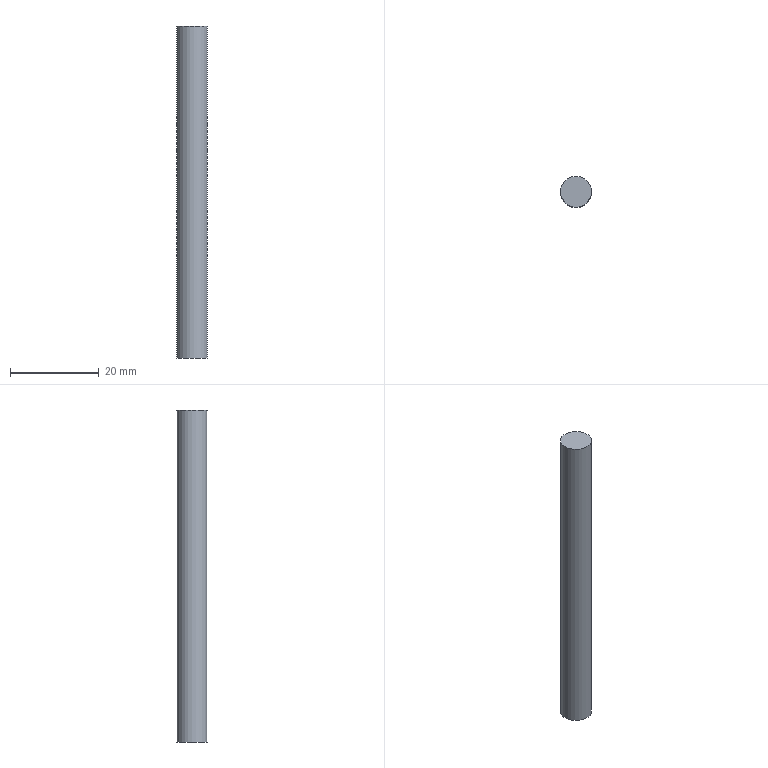Component | NX | SCREW_ROD_2 | 1 solid | 3 faces | box 6.99 x 6.99 x 75 mm | volume 2874 mm3 | plane 2 | cylinder 1 | commonest cylinder face diameters 6.985 x1
STEP:
#1=CARTESIAN_POINT('',(0.,0.,0.));
#2=DIRECTION('',(0.,0.,1.));
#3=DIRECTION('',(1.,0.,0.));
#4=AXIS2_PLACEMENT_3D('',#1,#2,#3);
#5=CARTESIAN_POINT('',(245.993,-0.,-15.));
#6=VERTEX_POINT('',#5);
#7=CARTESIAN_POINT('',(242.5,-0.,-15.));
#8=DIRECTION('',(0.,0.,-1.));
#9=DIRECTION('',(1.,0.,0.));
#10=AXIS2_PLACEMENT_3D('',#7,#8,#9);
#11=CIRCLE('',#10,3.493);
#12=CARTESIAN_POINT('',(242.5,-0.,-15.));
#13=DIRECTION('',(0.,0.,1.));
#14=DIRECTION('',(1.,0.,0.));
#15=AXIS2_PLACEMENT_3D('',#12,#13,#14);
#16=PLANE('',#15);
#17=CARTESIAN_POINT('',(3.493,0.));
#18=CARTESIAN_POINT('',(3.493,-6.049));
#19=CARTESIAN_POINT('',(-1.746,-3.025));
#20=CARTESIAN_POINT('',(-6.985,-0.));
#21=CARTESIAN_POINT('',(-1.746,3.025));
#22=CARTESIAN_POINT('',(3.493,6.049));
#23=CARTESIAN_POINT('',(3.493,0.));
#24=(BOUNDED_CURVE()B_SPLINE_CURVE(2,(#17,#18,#19,#20,#21,#22,#23),.UNSPECIFIED.,.T.,.F.)B_SPLINE_CURVE_WITH_KNOTS((1,2,2,2,2,1),(-2.094,0.,2.094,4.189,6.283,8.378),.UNSPECIFIED.)CURVE()GEOMETRIC_REPRESENTATION_ITEM()RATIONAL_B_SPLINE_CURVE((1.,0.5,1.,0.5,1.,0.5,1.))REPRESENTATION_ITEM(''));
#25=(GEOMETRIC_REPRESENTATION_CONTEXT(2)PARAMETRIC_REPRESENTATION_CONTEXT()REPRESENTATION_CONTEXT('',''));
#26=DEFINITIONAL_REPRESENTATION('',(#24),#25);
#27=PCURVE('',#16,#26);
#28=CARTESIAN_POINT('',(242.5,-0.,-90.));
#29=DIRECTION('',(0.,0.,1.));
#30=DIRECTION('',(1.,0.,0.));
#31=AXIS2_PLACEMENT_3D('',#28,#29,#30);
#32=CYLINDRICAL_SURFACE('',#31,3.493);
#33=CARTESIAN_POINT('',(6.283,75.));
#34=DIRECTION('',(-1.,0.));
#35=VECTOR('',#34,1.);
#36=LINE('',#33,#35);
#37=(GEOMETRIC_REPRESENTATION_CONTEXT(2)PARAMETRIC_REPRESENTATION_CONTEXT()REPRESENTATION_CONTEXT('',''));
#38=DEFINITIONAL_REPRESENTATION('',(#36),#37);
#39=PCURVE('',#32,#38);
#40=SURFACE_CURVE('',#11,(#27,#39),.PCURVE_S1.);
#41=EDGE_CURVE('',#6,#6,#40,.T.);
#42=ORIENTED_EDGE('',*,*,#41,.F.);
#43=EDGE_LOOP('',(#42));
#44=FACE_BOUND('',#43,.T.);
#45=ADVANCED_FACE('',(#44),#16,.T.);
#46=CARTESIAN_POINT('',(245.993,-0.,-90.));
#47=VERTEX_POINT('',#46);
#48=CARTESIAN_POINT('',(242.5,-0.,-90.));
#49=DIRECTION('',(0.,0.,1.));
#50=DIRECTION('',(1.,0.,0.));
#51=AXIS2_PLACEMENT_3D('',#48,#49,#50);
#52=CIRCLE('',#51,3.493);
#53=CARTESIAN_POINT('',(242.5,-0.,-90.));
#54=DIRECTION('',(0.,0.,-1.));
#55=DIRECTION('',(-1.,0.,0.));
#56=AXIS2_PLACEMENT_3D('',#53,#54,#55);
#57=PLANE('',#56);
#58=CARTESIAN_POINT('',(-3.493,0.));
#59=CARTESIAN_POINT('',(-3.493,6.049));
#60=CARTESIAN_POINT('',(1.746,3.025));
#61=CARTESIAN_POINT('',(6.985,0.));
#62=CARTESIAN_POINT('',(1.746,-3.025));
#63=CARTESIAN_POINT('',(-3.493,-6.049));
#64=CARTESIAN_POINT('',(-3.493,0.));
#65=(BOUNDED_CURVE()B_SPLINE_CURVE(2,(#58,#59,#60,#61,#62,#63,#64),.UNSPECIFIED.,.T.,.F.)B_SPLINE_CURVE_WITH_KNOTS((1,2,2,2,2,1),(-2.094,0.,2.094,4.189,6.283,8.378),.UNSPECIFIED.)CURVE()GEOMETRIC_REPRESENTATION_ITEM()RATIONAL_B_SPLINE_CURVE((1.,0.5,1.,0.5,1.,0.5,1.))REPRESENTATION_ITEM(''));
#66=(GEOMETRIC_REPRESENTATION_CONTEXT(2)PARAMETRIC_REPRESENTATION_CONTEXT()REPRESENTATION_CONTEXT('',''));
#67=DEFINITIONAL_REPRESENTATION('',(#65),#66);
#68=PCURVE('',#57,#67);
#69=CARTESIAN_POINT('',(0.,0.));
#70=DIRECTION('',(1.,0.));
#71=VECTOR('',#70,1.);
#72=LINE('',#69,#71);
#73=(GEOMETRIC_REPRESENTATION_CONTEXT(2)PARAMETRIC_REPRESENTATION_CONTEXT()REPRESENTATION_CONTEXT('',''));
#74=DEFINITIONAL_REPRESENTATION('',(#72),#73);
#75=PCURVE('',#32,#74);
#76=SURFACE_CURVE('',#52,(#68,#75),.PCURVE_S1.);
#77=EDGE_CURVE('',#47,#47,#76,.T.);
#78=ORIENTED_EDGE('',*,*,#77,.F.);
#79=EDGE_LOOP('',(#78));
#80=FACE_BOUND('',#79,.T.);
#81=ADVANCED_FACE('',(#80),#57,.T.);
#82=ORIENTED_EDGE('',*,*,#41,.T.);
#83=CARTESIAN_POINT('',(245.993,-0.,-90.));
#84=CARTESIAN_POINT('',(245.993,-0.,-15.));
#85=B_SPLINE_CURVE_WITH_KNOTS('',1,(#83,#84),.UNSPECIFIED.,.F.,.F.,(2,2),(0.,75.),.PIECEWISE_BEZIER_KNOTS.);
#86=CARTESIAN_POINT('',(0.,0.));
#87=DIRECTION('',(0.,1.));
#88=VECTOR('',#87,1.);
#89=LINE('',#86,#88);
#90=(GEOMETRIC_REPRESENTATION_CONTEXT(2)PARAMETRIC_REPRESENTATION_CONTEXT()REPRESENTATION_CONTEXT('',''));
#91=DEFINITIONAL_REPRESENTATION('',(#89),#90);
#92=PCURVE('',#32,#91);
#93=CARTESIAN_POINT('',(6.283,0.));
#94=DIRECTION('',(0.,1.));
#95=VECTOR('',#94,1.);
#96=LINE('',#93,#95);
#97=(GEOMETRIC_REPRESENTATION_CONTEXT(2)PARAMETRIC_REPRESENTATION_CONTEXT()REPRESENTATION_CONTEXT('',''));
#98=DEFINITIONAL_REPRESENTATION('',(#96),#97);
#99=PCURVE('',#32,#98);
#100=SEAM_CURVE('',#85,(#92,#99),.PCURVE_S1.);
#101=EDGE_CURVE('',#47,#6,#100,.T.);
#102=ORIENTED_EDGE('',*,*,#101,.F.);
#103=ORIENTED_EDGE('',*,*,#77,.T.);
#104=ORIENTED_EDGE('',*,*,#101,.T.);
#105=EDGE_LOOP('',(#82,#102,#103,#104));
#106=FACE_BOUND('',#105,.T.);
#107=ADVANCED_FACE('',(#106),#32,.T.);
#108=CLOSED_SHELL('',(#45,#81,#107));
#109=MANIFOLD_SOLID_BREP('',#108);
#110=(LENGTH_UNIT()NAMED_UNIT(*)SI_UNIT(.MILLI.,.METRE.));
#111=UNCERTAINTY_MEASURE_WITH_UNIT(LENGTH_MEASURE(0.00001),#110,'','');
#112=(NAMED_UNIT(*)PLANE_ANGLE_UNIT()SI_UNIT($,.RADIAN.));
#113=(NAMED_UNIT(*)SI_UNIT($,.STERADIAN.)SOLID_ANGLE_UNIT());
#114=(GEOMETRIC_REPRESENTATION_CONTEXT(3)GLOBAL_UNCERTAINTY_ASSIGNED_CONTEXT((#111))GLOBAL_UNIT_ASSIGNED_CONTEXT((#110,#112,#113))REPRESENTATION_CONTEXT('',''));
#115=ADVANCED_BREP_SHAPE_REPRESENTATION('',(#4,#109),#114);